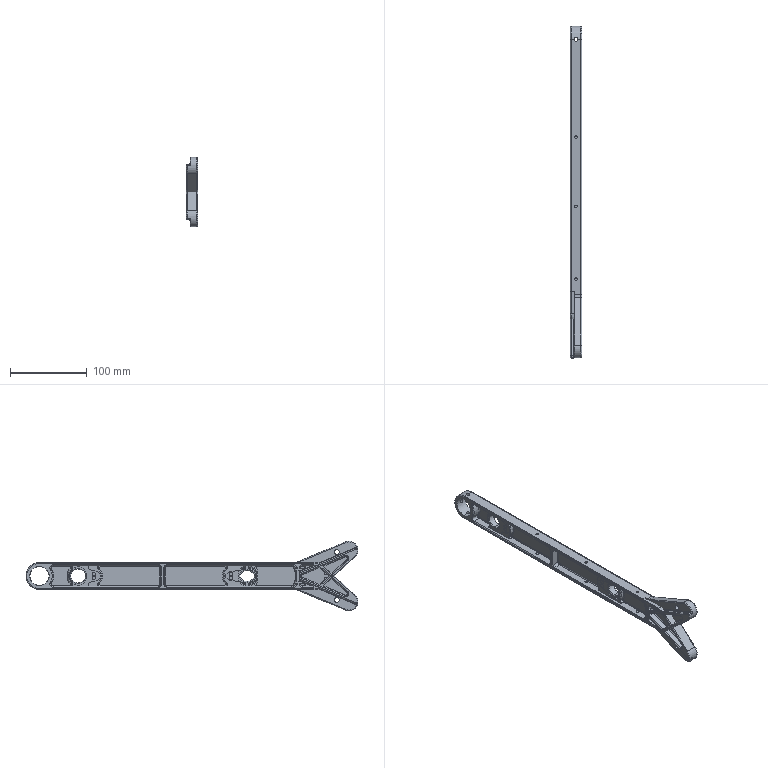CAM job | Mastercam | mm | 2 operations | part box 15 x 431.82 x 90.58
1. Drill/Counterbore | 7 - 4 倒角刀
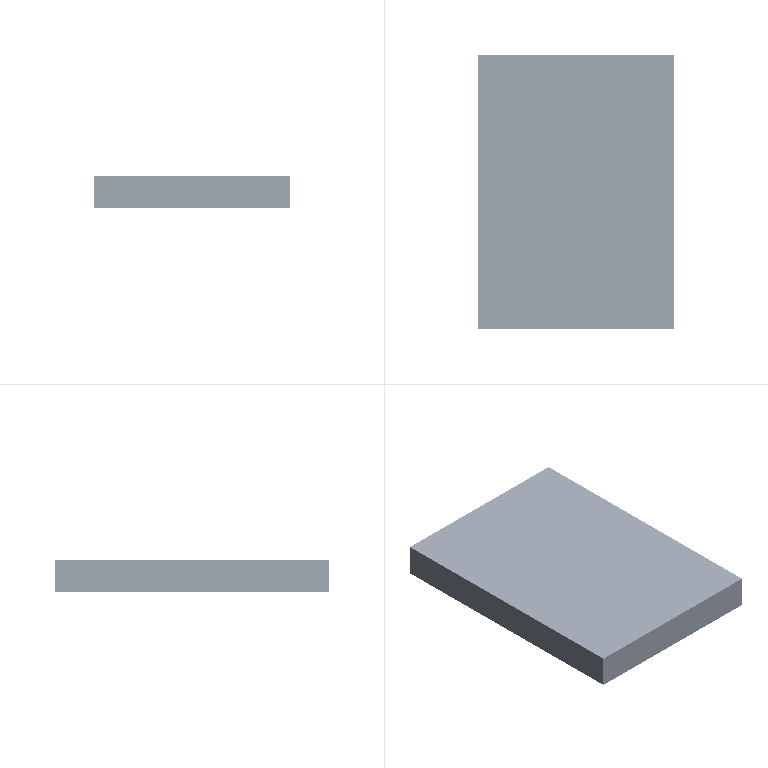2. Drill/Counterbore | 7 - 4 倒角刀